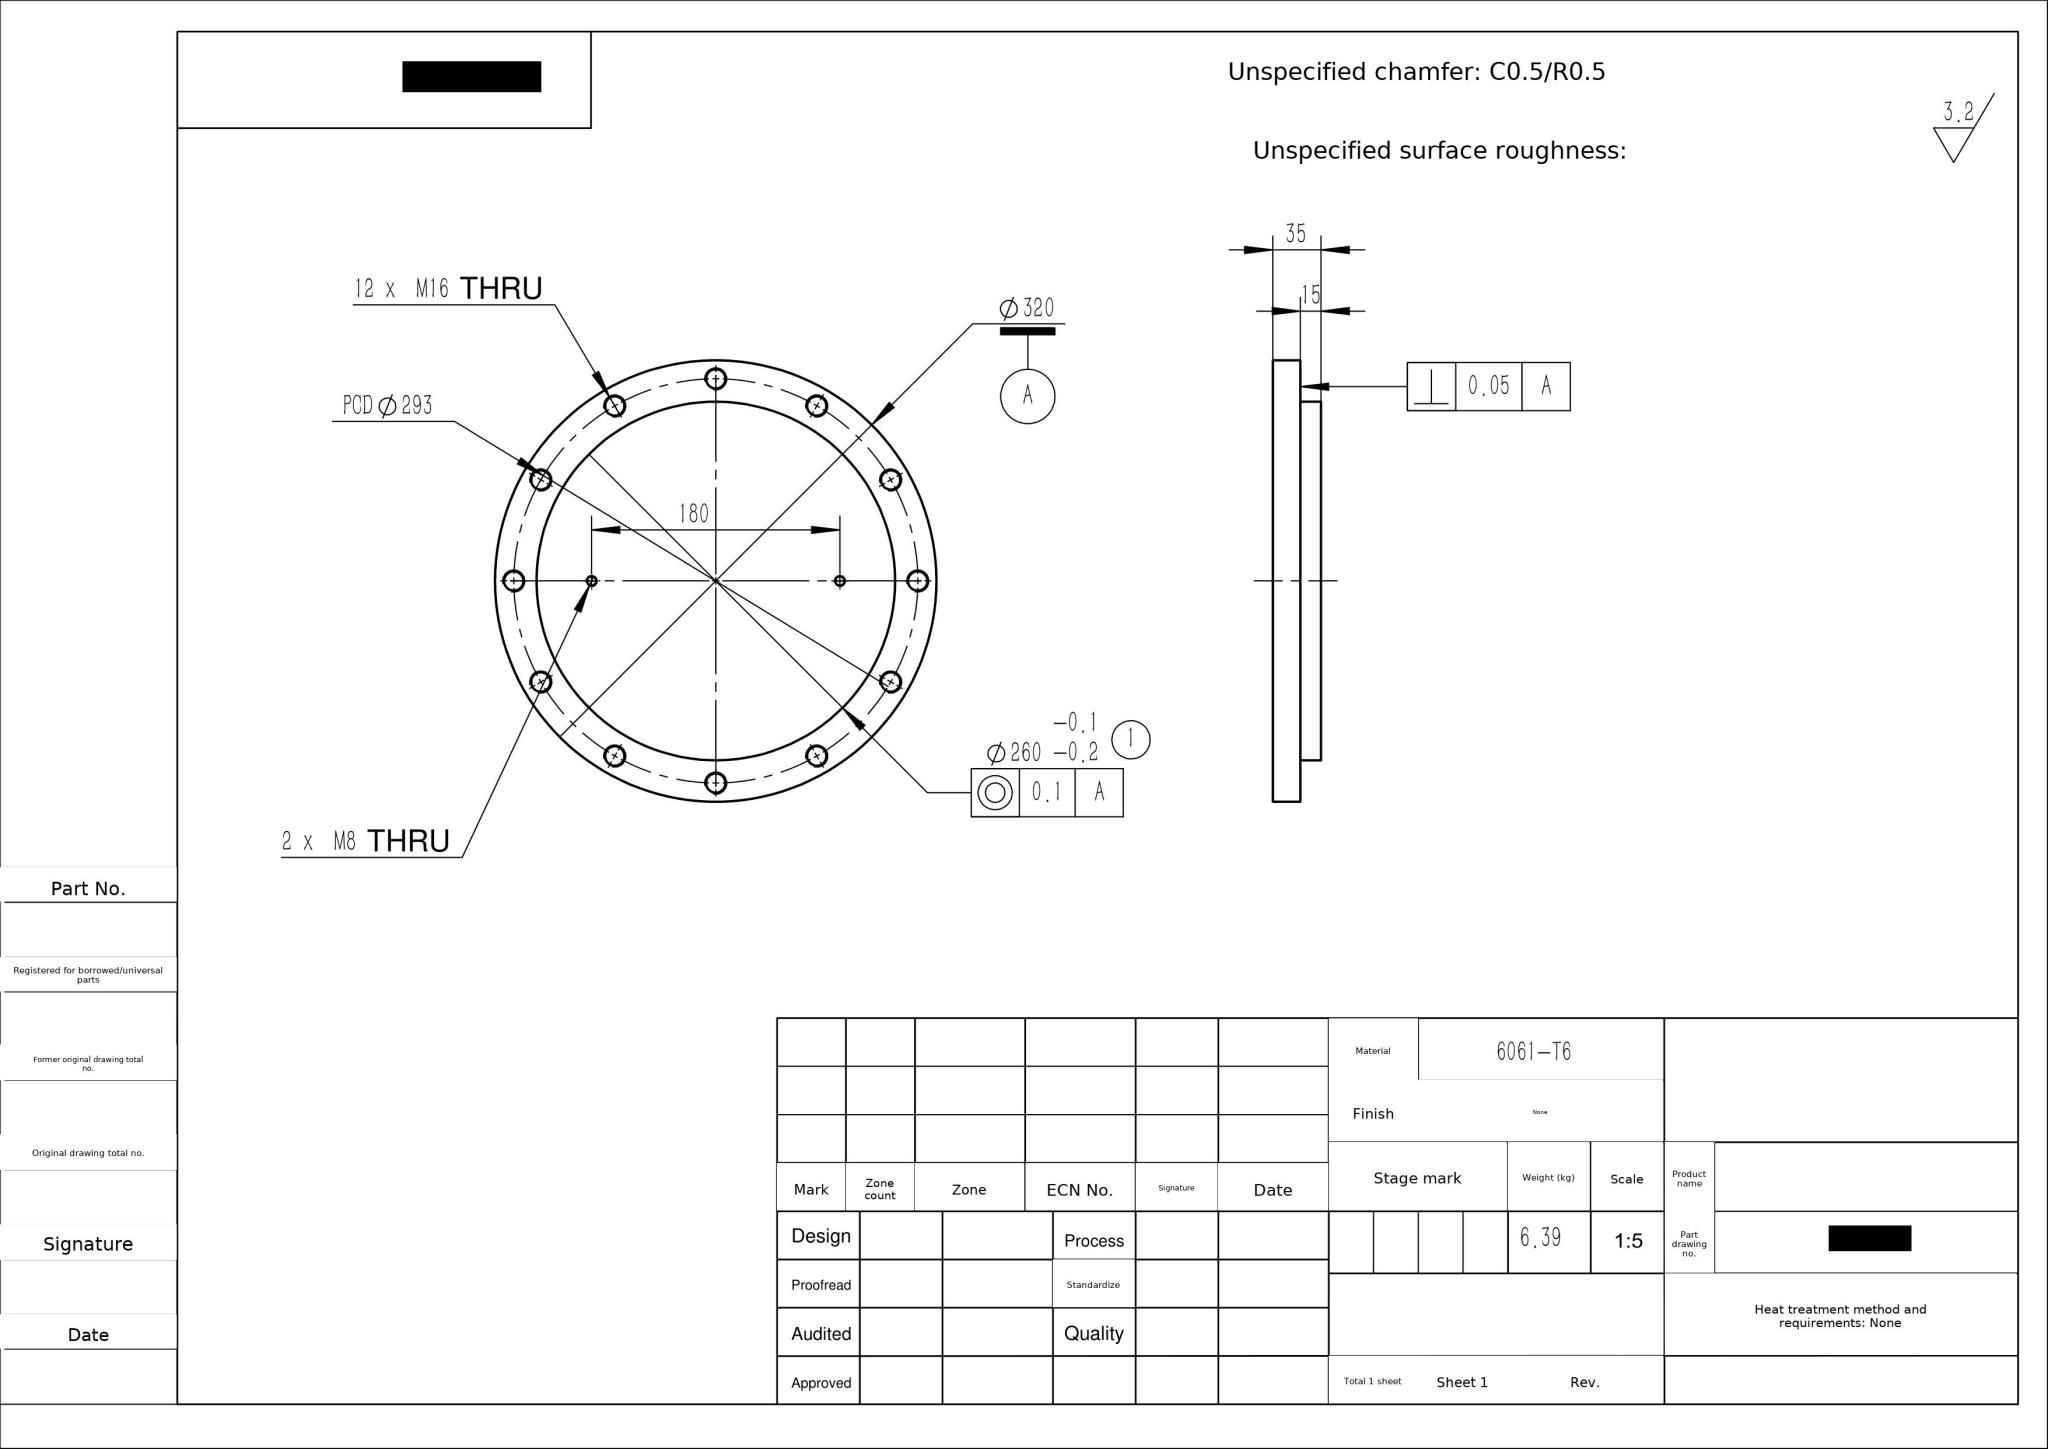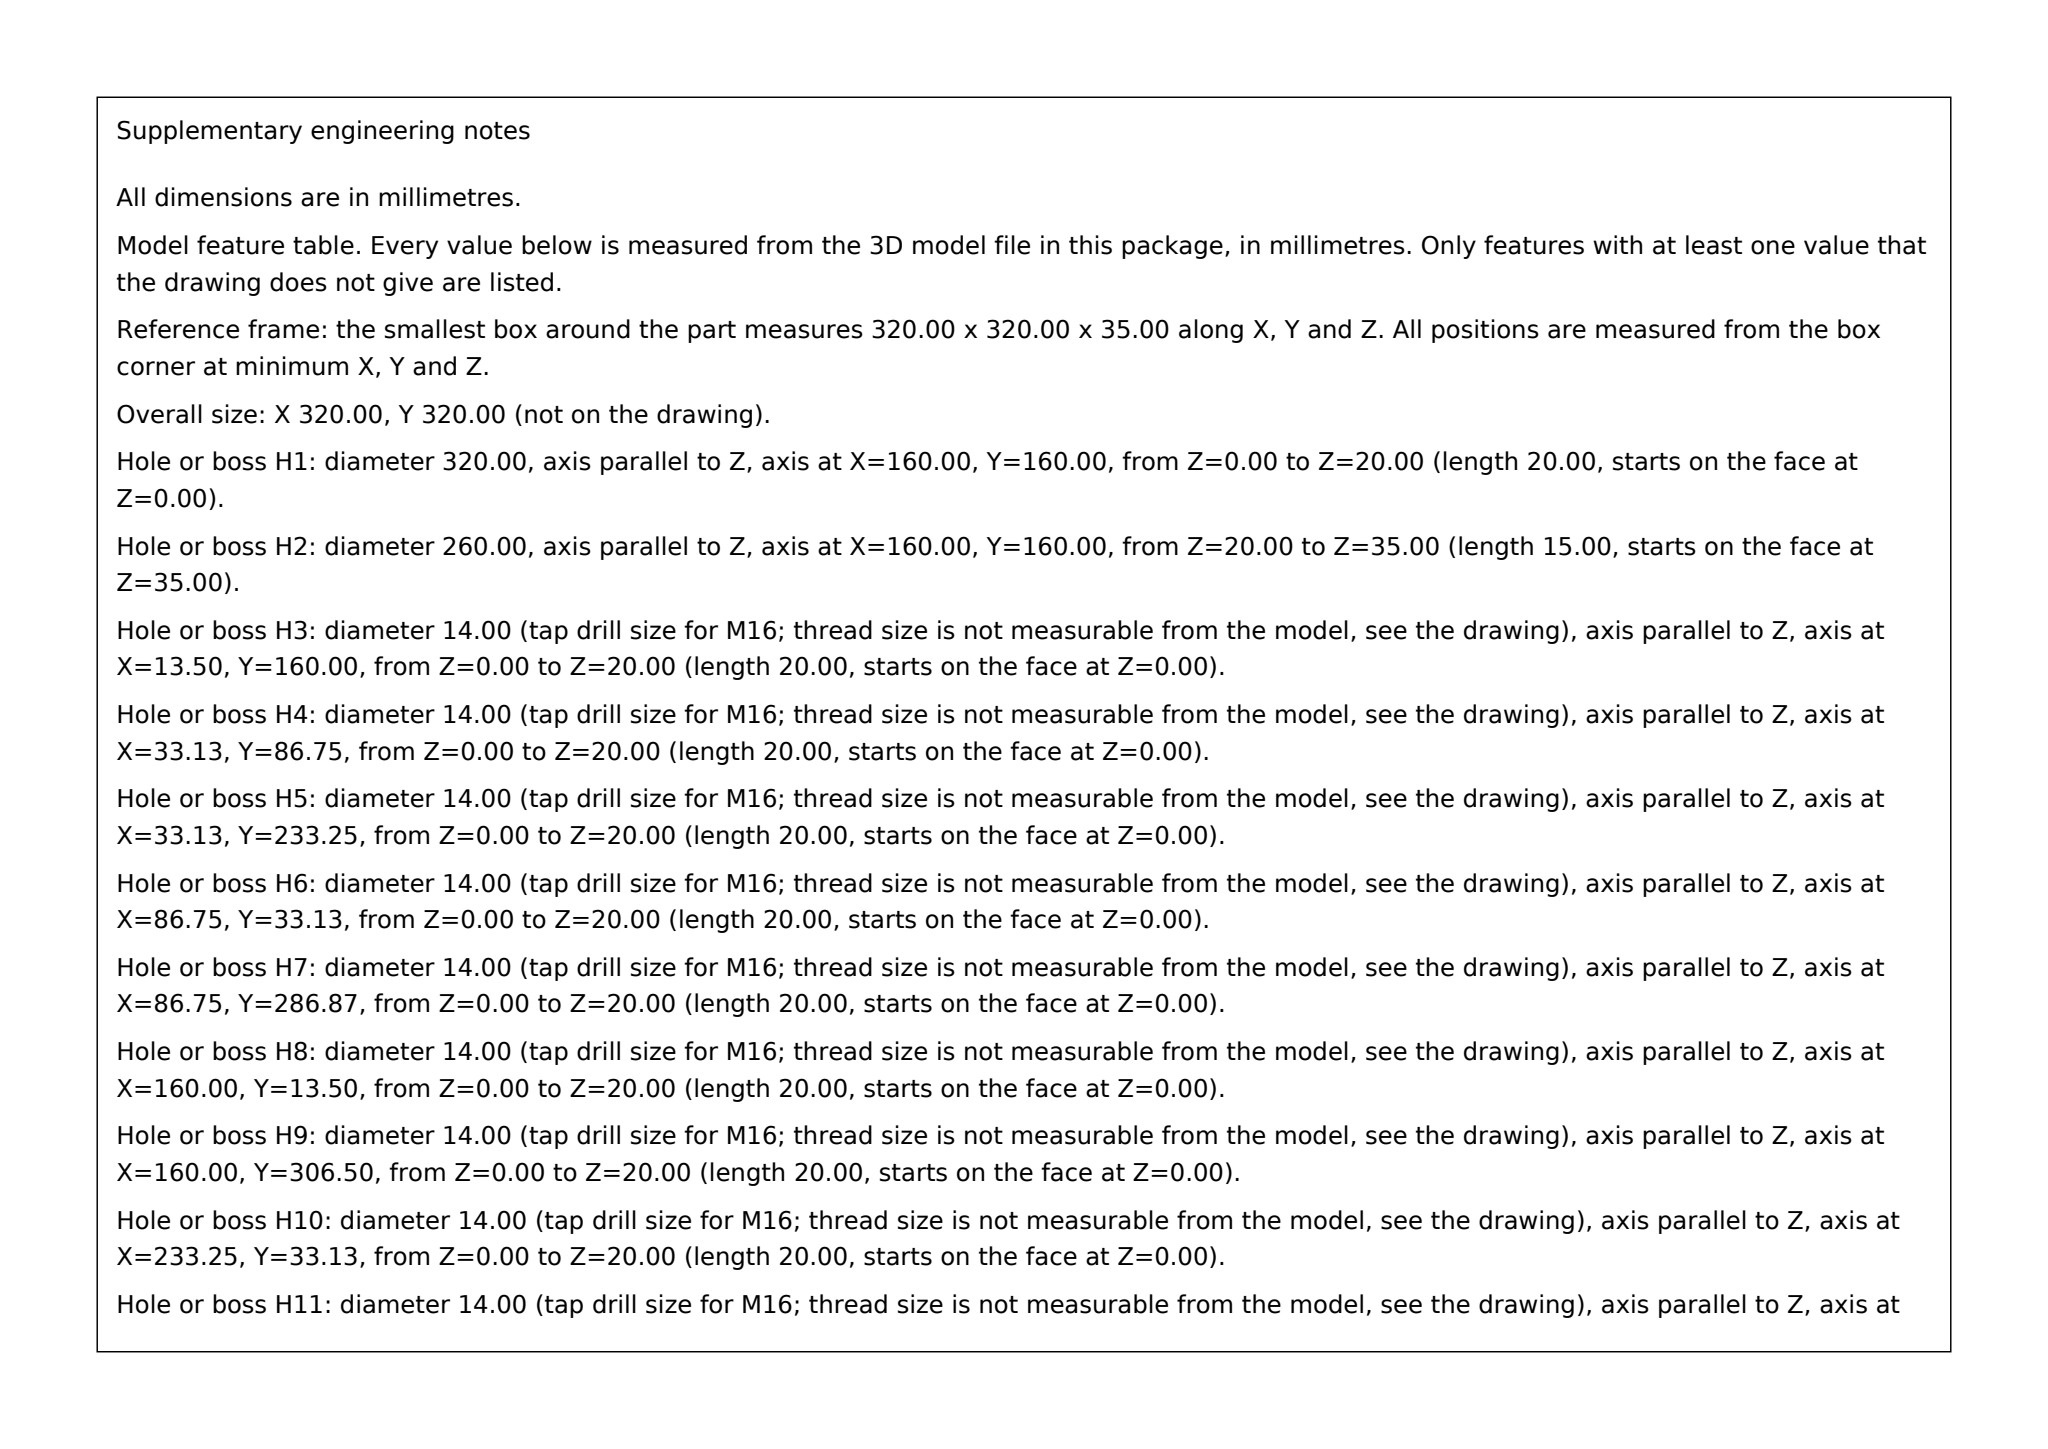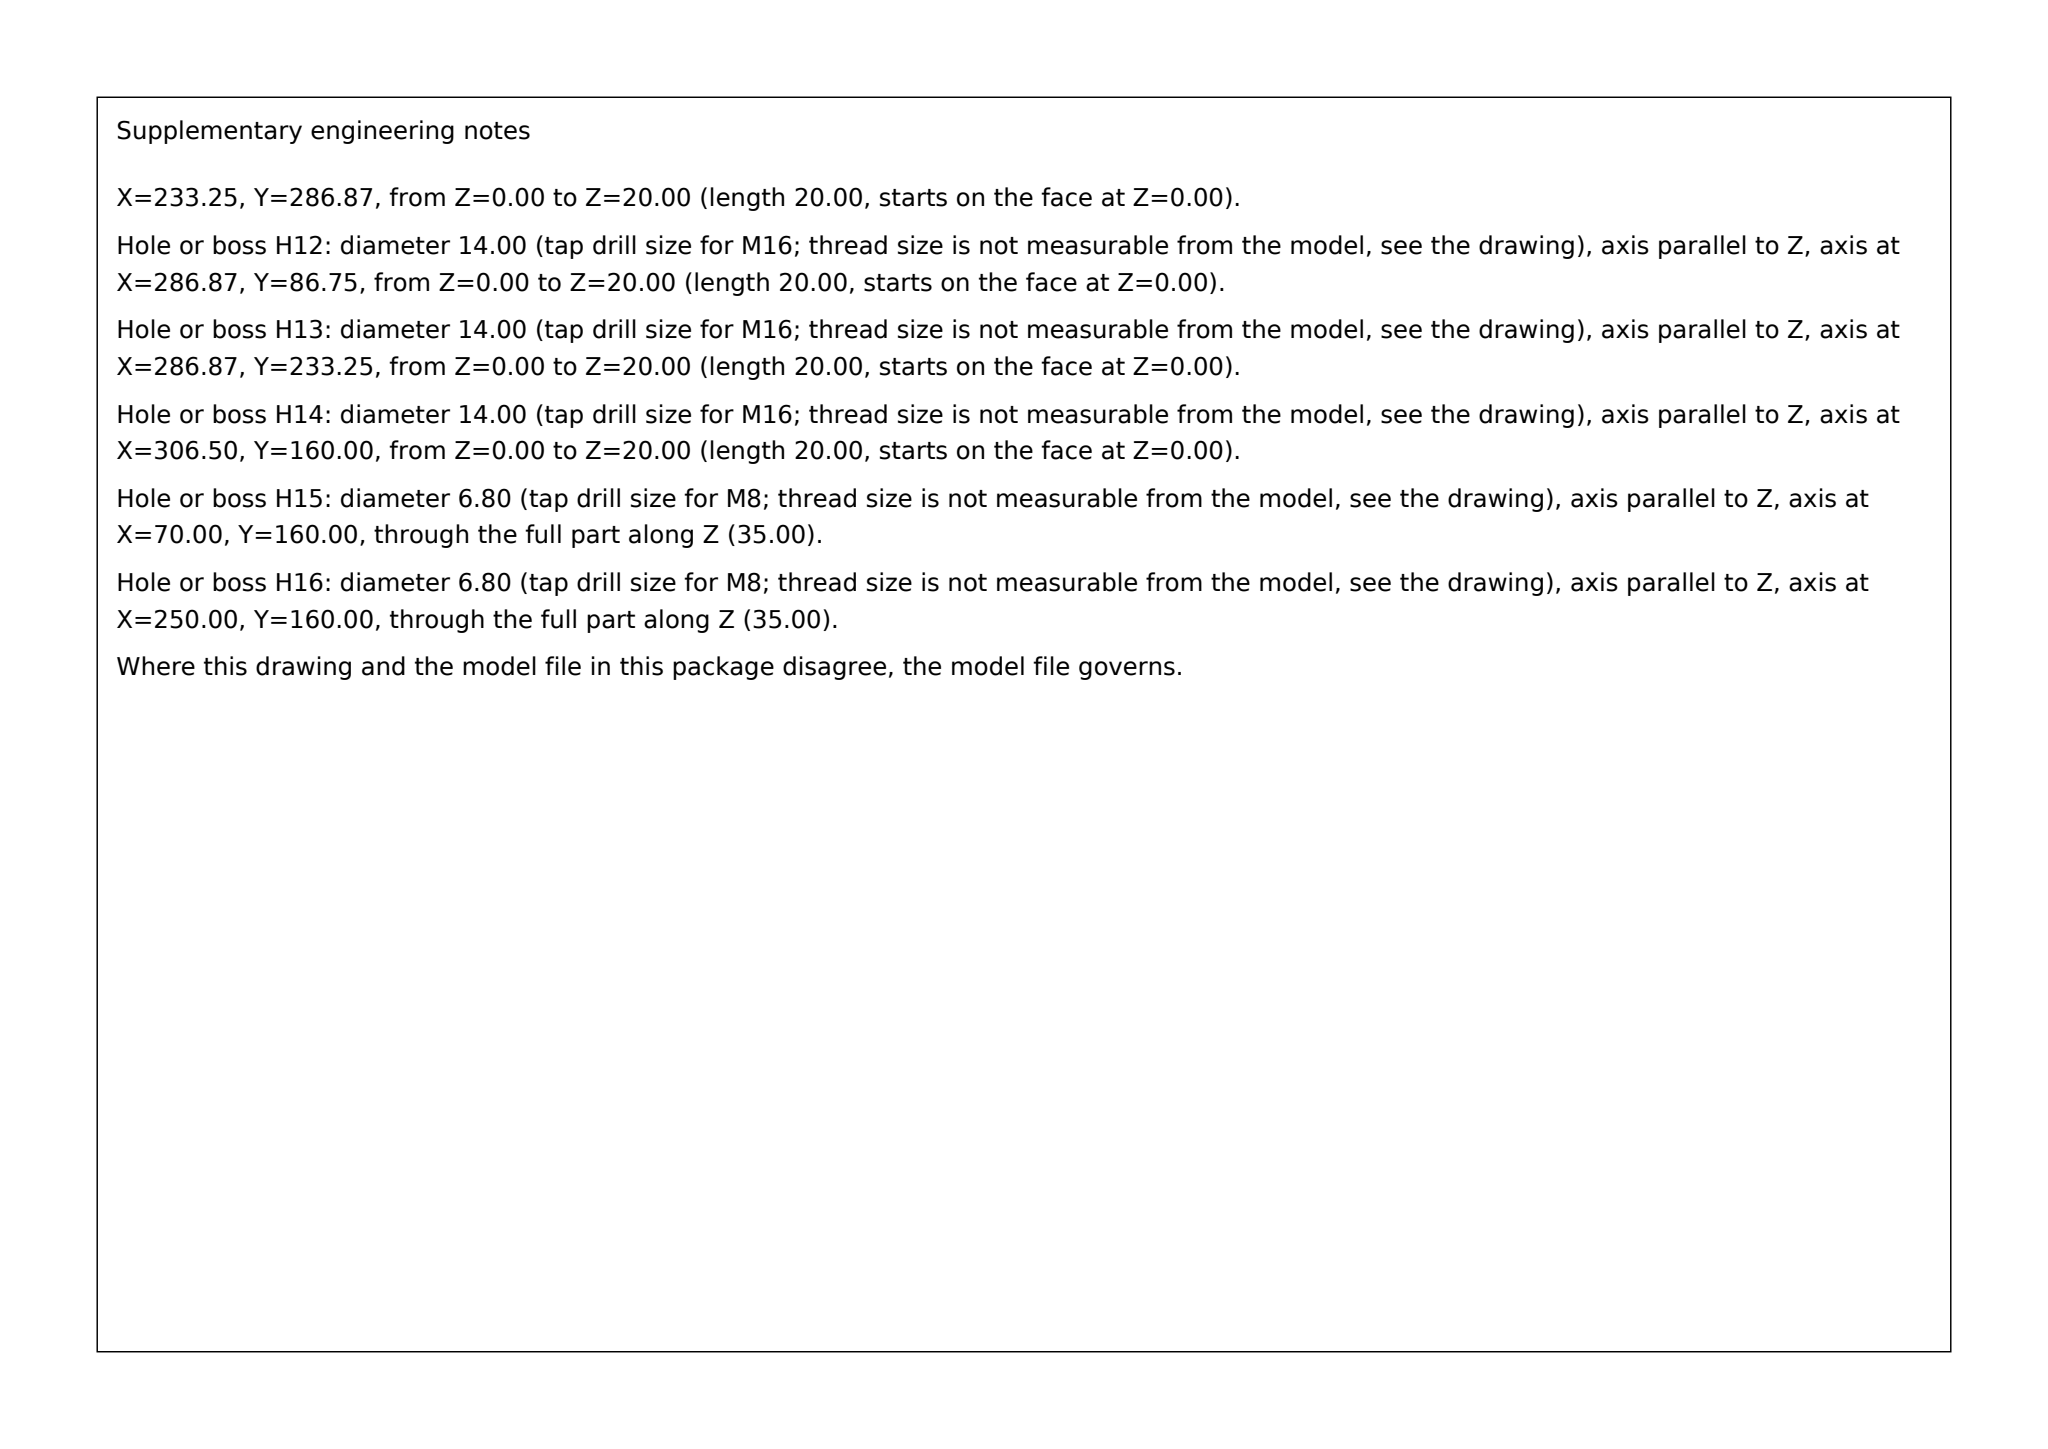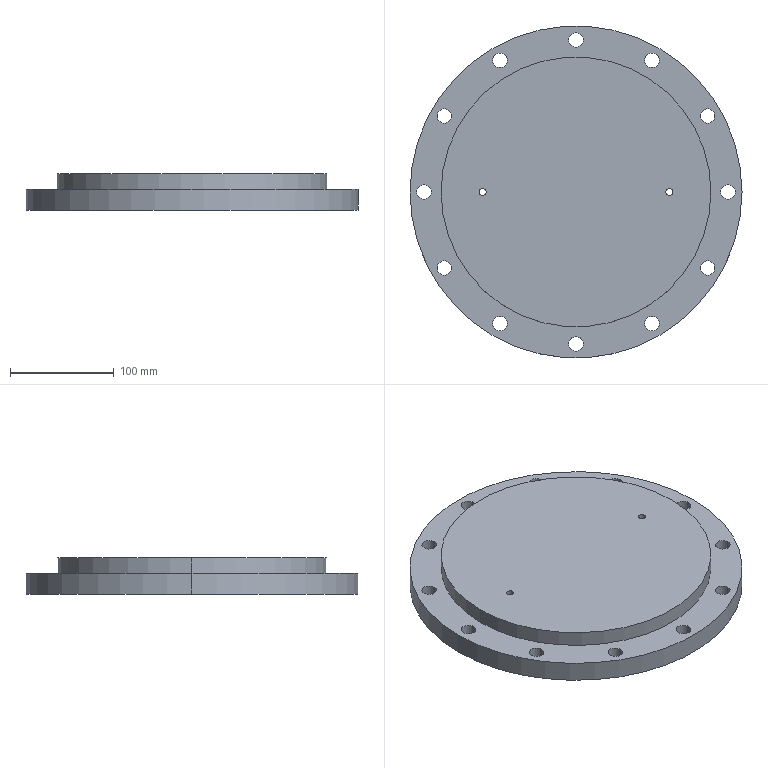Part | SolidWorks | mm | material 6061-T6 | 1 solid | 35 faces | box 320 x 320 x 35 mm | volume 2365402 mm3 | cylinder 32 | plane 3 | commonest cylinder face diameters 14 x24 6.8 x4 320 x2 260 x2
build123d program:
from build123d import *

# Parameters (mm, degrees)
SKETCH1_R           = 130
BOSS_EXTRUDE1_DEPTH = 15
SKETCH2_R           = 160
BOSS_EXTRUDE2_DEPTH = 20
M16_TAPPED_HOLE1_D  = 14
CIRPATTERN1_COUNT   = 12
M8_TAPPED_HOLE1_D   = 6.8


with BuildPart() as part:
    # Sketch1 → Boss-Extrude1 (new body)
    with BuildSketch(Plane.XY):
        Circle(SKETCH1_R)
    extrude(amount=BOSS_EXTRUDE1_DEPTH)

    # Sketch2 → Boss-Extrude2 (add)
    with BuildSketch(Plane(origin=(0, 0, 0), x_dir=(-1, 0, 0), z_dir=(0, 0, -1))):
        Circle(SKETCH2_R)
    extrude(amount=BOSS_EXTRUDE2_DEPTH)

    # M16 Tapped Hole1 (through all)
    with Locations(Plane(origin=(0, 0, -20), x_dir=(-1, 0, 0), z_dir=(0, 0, -1))):
        with Locations((0, -146.5)):
            m16_tapped_hole1 = Hole(M16_TAPPED_HOLE1_D / 2)

    # CirPattern1: M16 Tapped Hole1 ×12 about axis
    cirpattern1_axis = Axis((0, 0, 0), (0, 0, 1))
    for i in range(1, CIRPATTERN1_COUNT):
        add(m16_tapped_hole1.rotate(cirpattern1_axis, i * 360 / CIRPATTERN1_COUNT), mode=Mode.SUBTRACT)

    # M8 Tapped Hole1 (through all)
    with Locations(Plane(origin=(0, 0, -20), x_dir=(-1, 0, 0), z_dir=(0, 0, -1))):
        with Locations((90, 0), (-90, 0)):
            Hole(M8_TAPPED_HOLE1_D / 2)


solid = part.part